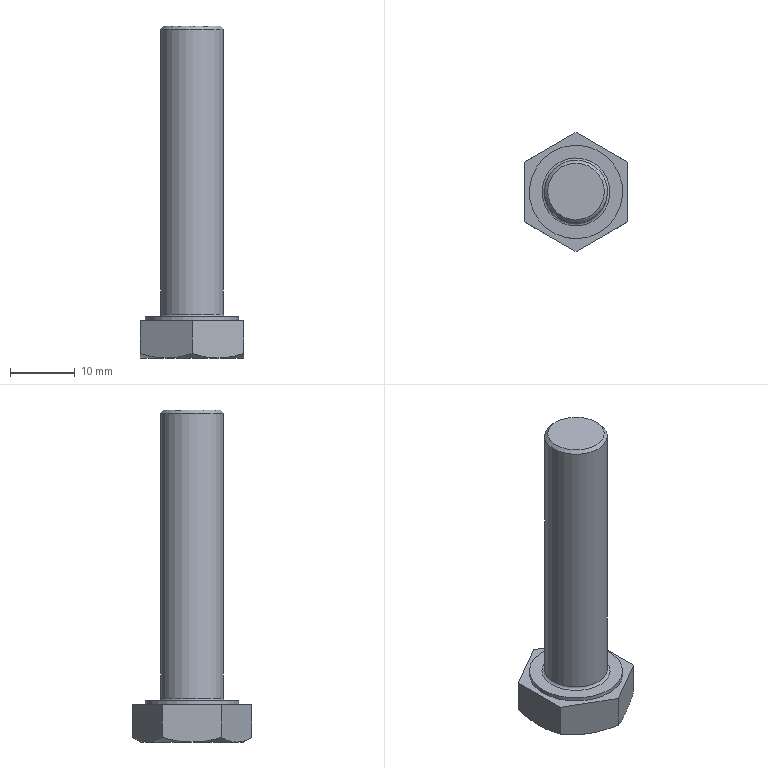Component | NX | GB-T5782-2000_M10X45 | 1 solid | 20 faces | volume 4725 mm3 | plane 10 | cone 7 | cylinder 2 | torus 1 | commonest cylinder face diameters 14.47 x1 9.732 x1